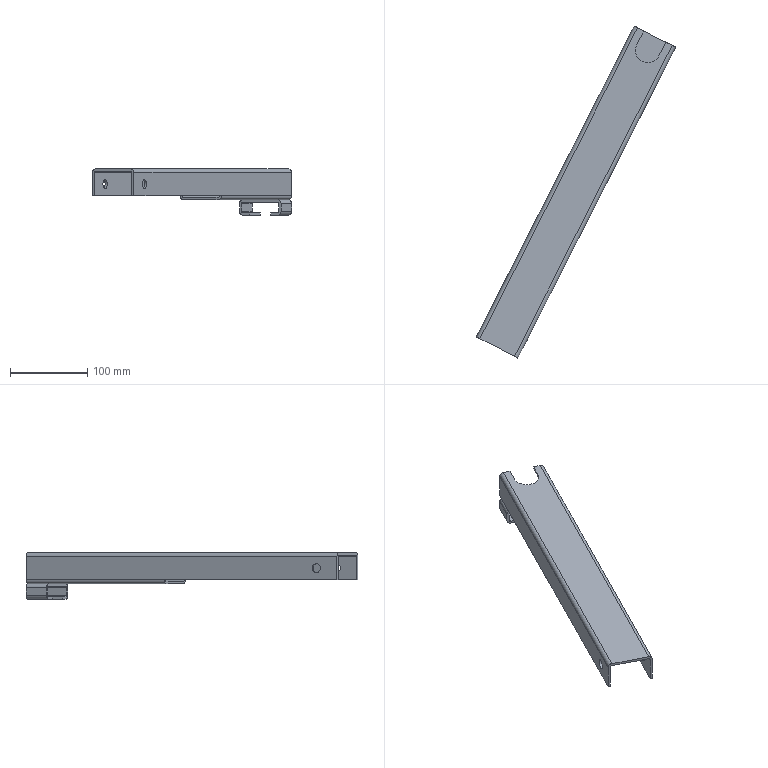Component | SolidWorks | ScribingMechanismAssembly-1_FilmBracketTube-1 | 2 solids | 50 faces | volume 206216 mm3 | plane 29 | cylinder 21 | commonest cylinder face diameters 10 x8 4 x8 12 x4 32 x1